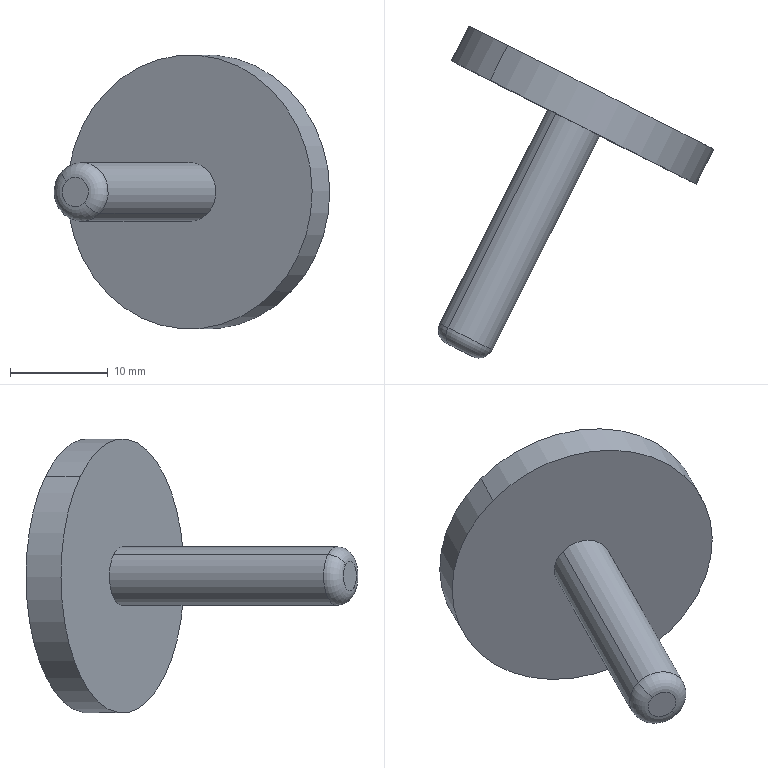Component | SolidWorks | Part15-1 | 2 solids | 10 faces | box 28.16 x 33.93 x 28 mm | volume 3190 mm3 | cylinder 4 | plane 4 | torus 2 | commonest cylinder face diameters 6 x2 28 x2
STEP:
#1=COLOUR_RGB('',0.7922,0.8196,0.9333);
#2=FILL_AREA_STYLE_COLOUR('',#1);
#3=FILL_AREA_STYLE('',(#2));
#4=SURFACE_STYLE_FILL_AREA(#3);
#5=SURFACE_SIDE_STYLE('',(#4));
#6=SURFACE_STYLE_USAGE(.BOTH.,#5);
#7=PRESENTATION_STYLE_ASSIGNMENT((#6));
#8=CARTESIAN_POINT('',(1.257,1.983,-0.3626));
#9=VERTEX_POINT('',#8);
#10=CARTESIAN_POINT('',(0.5828,2.322,0.4413));
#11=VERTEX_POINT('',#10);
#12=CARTESIAN_POINT('',(0.9197,2.152,0.03937));
#13=DIRECTION('',(0.4496,0.8932,-0.));
#14=DIRECTION('',(0.6112,-0.3076,-0.7292));
#15=AXIS2_PLACEMENT_3D('',#12,#13,#14);
#16=CIRCLE('',#15,0.5512);
#17=EDGE_CURVE('',#9,#11,#16,.T.);
#18=ORIENTED_EDGE('',*,*,#17,.F.);
#19=CARTESIAN_POINT('',(1.186,1.842,-0.3626));
#20=VERTEX_POINT('',#19);
#21=CARTESIAN_POINT('',(1.257,1.983,-0.3626));
#22=DIRECTION('',(-0.4496,-0.8932,0.));
#23=VECTOR('',#22,39.37);
#24=LINE('',#21,#23);
#25=EDGE_CURVE('',#9,#20,#24,.T.);
#26=ORIENTED_EDGE('',*,*,#25,.T.);
#27=CARTESIAN_POINT('',(0.512,2.181,0.4413));
#28=VERTEX_POINT('',#27);
#29=CARTESIAN_POINT('',(0.8489,2.012,0.03937));
#30=DIRECTION('',(0.4496,0.8932,-0.));
#31=DIRECTION('',(0.6112,-0.3076,-0.7292));
#32=AXIS2_PLACEMENT_3D('',#29,#30,#31);
#33=CIRCLE('',#32,0.5512);
#34=EDGE_CURVE('',#20,#28,#33,.T.);
#35=ORIENTED_EDGE('',*,*,#34,.T.);
#36=CARTESIAN_POINT('',(0.5828,2.322,0.4413));
#37=DIRECTION('',(-0.4496,-0.8932,0.));
#38=VECTOR('',#37,39.37);
#39=LINE('',#36,#38);
#40=EDGE_CURVE('',#11,#28,#39,.T.);
#41=ORIENTED_EDGE('',*,*,#40,.F.);
#42=EDGE_LOOP('',(#18,#26,#35,#41));
#43=FACE_OUTER_BOUND('',#42,.T.);
#44=CARTESIAN_POINT('',(0.9197,2.152,0.03937));
#45=DIRECTION('',(-0.4496,-0.8932,0.));
#46=DIRECTION('',(-0.6112,0.3076,0.7292));
#47=AXIS2_PLACEMENT_3D('',#44,#45,#46);
#48=CYLINDRICAL_SURFACE('',#47,0.5512);
#49=ADVANCED_FACE('',(#43),#48,.T.);
#50=CARTESIAN_POINT('',(0.8489,2.012,0.03937));
#51=DIRECTION('',(0.4496,0.8932,-0.));
#52=DIRECTION('',(0.6112,-0.3076,-0.7292));
#53=AXIS2_PLACEMENT_3D('',#50,#51,#52);
#54=CIRCLE('',#53,0.5512);
#55=EDGE_CURVE('',#28,#20,#54,.T.);
#56=ORIENTED_EDGE('',*,*,#55,.F.);
#57=ORIENTED_EDGE('',*,*,#34,.F.);
#58=EDGE_LOOP('',(#56,#57));
#59=FACE_OUTER_BOUND('',#58,.T.);
#60=CARTESIAN_POINT('',(0.8489,2.012,0.03937));
#61=DIRECTION('',(0.4496,0.8932,-0.));
#62=DIRECTION('',(0.6514,-0.3278,0.6843));
#63=AXIS2_PLACEMENT_3D('',#60,#61,#62);
#64=PLANE('',#63);
#65=ADVANCED_FACE('',(#59),#64,.F.);
#66=CARTESIAN_POINT('',(0.9197,2.152,0.03937));
#67=DIRECTION('',(0.4496,0.8932,-0.));
#68=DIRECTION('',(0.6112,-0.3076,-0.7292));
#69=AXIS2_PLACEMENT_3D('',#66,#67,#68);
#70=CIRCLE('',#69,0.5512);
#71=EDGE_CURVE('',#11,#9,#70,.T.);
#72=ORIENTED_EDGE('',*,*,#71,.T.);
#73=ORIENTED_EDGE('',*,*,#17,.T.);
#74=EDGE_LOOP('',(#72,#73));
#75=FACE_OUTER_BOUND('',#74,.T.);
#76=CARTESIAN_POINT('',(0.9197,2.152,0.03937));
#77=DIRECTION('',(0.4496,0.8932,-0.));
#78=DIRECTION('',(0.6514,-0.3278,0.6843));
#79=AXIS2_PLACEMENT_3D('',#76,#77,#78);
#80=PLANE('',#79);
#81=ADVANCED_FACE('',(#75),#80,.T.);
#82=ORIENTED_EDGE('',*,*,#25,.F.);
#83=ORIENTED_EDGE('',*,*,#71,.F.);
#84=ORIENTED_EDGE('',*,*,#40,.T.);
#85=ORIENTED_EDGE('',*,*,#55,.T.);
#86=EDGE_LOOP('',(#82,#83,#84,#85));
#87=FACE_OUTER_BOUND('',#86,.T.);
#88=CARTESIAN_POINT('',(0.9197,2.152,0.03937));
#89=DIRECTION('',(-0.4496,-0.8932,0.));
#90=DIRECTION('',(-0.6112,0.3076,0.7292));
#91=AXIS2_PLACEMENT_3D('',#88,#89,#90);
#92=CYLINDRICAL_SURFACE('',#91,0.5512);
#93=ADVANCED_FACE('',(#87),#92,.T.);
#94=CLOSED_SHELL('',(#49,#65,#81,#93));
#95=MANIFOLD_SOLID_BREP('',#94);
#96=STYLED_ITEM('',(#7),#95);
#97=PRESENTATION_LAYER_ASSIGNMENT('','',(#96));
#98=COLOUR_RGB('',0.7922,0.8196,0.9333);
#99=FILL_AREA_STYLE_COLOUR('',#98);
#100=FILL_AREA_STYLE('',(#99));
#101=SURFACE_STYLE_FILL_AREA(#100);
#102=SURFACE_SIDE_STYLE('',(#101));
#103=SURFACE_STYLE_USAGE(.BOTH.,#102);
#104=PRESENTATION_STYLE_ASSIGNMENT((#103));
#105=CARTESIAN_POINT('',(0.4874,1.114,-0.04676));
#106=VERTEX_POINT('',#105);
#107=CARTESIAN_POINT('',(0.343,1.186,0.1255));
#108=VERTEX_POINT('',#107);
#109=CARTESIAN_POINT('',(0.4152,1.15,0.03937));
#110=DIRECTION('',(0.4496,0.8932,-0.));
#111=DIRECTION('',(-0.6112,0.3076,0.7292));
#112=AXIS2_PLACEMENT_3D('',#109,#110,#111);
#113=CIRCLE('',#112,0.1181);
#114=EDGE_CURVE('',#106,#108,#113,.T.);
#115=ORIENTED_EDGE('',*,*,#114,.T.);
#116=CARTESIAN_POINT('',(0.7767,2.048,0.1255));
#117=VERTEX_POINT('',#116);
#118=CARTESIAN_POINT('',(0.3165,1.134,0.1255));
#119=DIRECTION('',(0.4496,0.8932,-0.));
#120=VECTOR('',#119,39.37);
#121=LINE('',#118,#120);
#122=EDGE_CURVE('',#108,#117,#121,.T.);
#123=ORIENTED_EDGE('',*,*,#122,.T.);
#124=CARTESIAN_POINT('',(0.9211,1.975,-0.04676));
#125=VERTEX_POINT('',#124);
#126=CARTESIAN_POINT('',(0.8489,2.012,0.03937));
#127=DIRECTION('',(-0.4496,-0.8932,0.));
#128=DIRECTION('',(-0.6112,0.3076,0.7292));
#129=AXIS2_PLACEMENT_3D('',#126,#127,#128);
#130=CIRCLE('',#129,0.1181);
#131=EDGE_CURVE('',#117,#125,#130,.T.);
#132=ORIENTED_EDGE('',*,*,#131,.T.);
#133=CARTESIAN_POINT('',(0.4609,1.061,-0.04676));
#134=DIRECTION('',(0.4496,0.8932,-0.));
#135=VECTOR('',#134,39.37);
#136=LINE('',#133,#135);
#137=EDGE_CURVE('',#106,#125,#136,.T.);
#138=ORIENTED_EDGE('',*,*,#137,.F.);
#139=EDGE_LOOP('',(#115,#123,#132,#138));
#140=FACE_OUTER_BOUND('',#139,.T.);
#141=CARTESIAN_POINT('',(0.3887,1.097,0.03937));
#142=DIRECTION('',(0.4496,0.8932,-0.));
#143=DIRECTION('',(0.6112,-0.3076,-0.7292));
#144=AXIS2_PLACEMENT_3D('',#141,#142,#143);
#145=CYLINDRICAL_SURFACE('',#144,0.1181);
#146=ADVANCED_FACE('',(#140),#145,.T.);
#147=ORIENTED_EDGE('',*,*,#114,.F.);
#148=CARTESIAN_POINT('',(0.4248,1.079,-0.003695));
#149=VERTEX_POINT('',#148);
#150=CARTESIAN_POINT('',(0.4513,1.132,-0.003695));
#151=DIRECTION('',(-0.6514,0.3278,-0.6843));
#152=DIRECTION('',(-0.7243,0.,0.6895));
#153=AXIS2_PLACEMENT_3D('',#150,#151,#152);
#154=CIRCLE('',#153,0.05906);
#155=EDGE_CURVE('',#106,#149,#154,.T.);
#156=ORIENTED_EDGE('',*,*,#155,.T.);
#157=CARTESIAN_POINT('',(0.3526,1.115,0.08243));
#158=VERTEX_POINT('',#157);
#159=CARTESIAN_POINT('',(0.3887,1.097,0.03937));
#160=DIRECTION('',(-0.4496,-0.8932,0.));
#161=DIRECTION('',(-0.6112,0.3076,0.7292));
#162=AXIS2_PLACEMENT_3D('',#159,#160,#161);
#163=CIRCLE('',#162,0.05906);
#164=EDGE_CURVE('',#158,#149,#163,.T.);
#165=ORIENTED_EDGE('',*,*,#164,.F.);
#166=CARTESIAN_POINT('',(0.3791,1.168,0.08243));
#167=DIRECTION('',(0.6514,-0.3278,0.6843));
#168=DIRECTION('',(0.7243,0.,-0.6895));
#169=AXIS2_PLACEMENT_3D('',#166,#167,#168);
#170=CIRCLE('',#169,0.05906);
#171=EDGE_CURVE('',#108,#158,#170,.T.);
#172=ORIENTED_EDGE('',*,*,#171,.F.);
#173=EDGE_LOOP('',(#147,#156,#165,#172));
#174=FACE_OUTER_BOUND('',#173,.T.);
#175=CARTESIAN_POINT('',(0.4152,1.15,0.03937));
#176=DIRECTION('',(-0.4496,-0.8932,0.));
#177=DIRECTION('',(-0.6112,0.3076,0.7292));
#178=AXIS2_PLACEMENT_3D('',#175,#176,#177);
#179=TOROIDAL_SURFACE('',#178,0.05906,0.05906);
#180=ADVANCED_FACE('',(#174),#179,.T.);
#181=ORIENTED_EDGE('',*,*,#155,.F.);
#182=CARTESIAN_POINT('',(0.4152,1.15,0.03937));
#183=DIRECTION('',(0.4496,0.8932,-0.));
#184=DIRECTION('',(-0.6112,0.3076,0.7292));
#185=AXIS2_PLACEMENT_3D('',#182,#183,#184);
#186=CIRCLE('',#185,0.1181);
#187=EDGE_CURVE('',#108,#106,#186,.T.);
#188=ORIENTED_EDGE('',*,*,#187,.F.);
#189=ORIENTED_EDGE('',*,*,#171,.T.);
#190=CARTESIAN_POINT('',(0.3887,1.097,0.03937));
#191=DIRECTION('',(-0.4496,-0.8932,0.));
#192=DIRECTION('',(-0.6112,0.3076,0.7292));
#193=AXIS2_PLACEMENT_3D('',#190,#191,#192);
#194=CIRCLE('',#193,0.05906);
#195=EDGE_CURVE('',#149,#158,#194,.T.);
#196=ORIENTED_EDGE('',*,*,#195,.F.);
#197=EDGE_LOOP('',(#181,#188,#189,#196));
#198=FACE_OUTER_BOUND('',#197,.T.);
#199=CARTESIAN_POINT('',(0.4152,1.15,0.03937));
#200=DIRECTION('',(-0.4496,-0.8932,0.));
#201=DIRECTION('',(-0.6112,0.3076,0.7292));
#202=AXIS2_PLACEMENT_3D('',#199,#200,#201);
#203=TOROIDAL_SURFACE('',#202,0.05906,0.05906);
#204=ADVANCED_FACE('',(#198),#203,.T.);
#205=CARTESIAN_POINT('',(0.8489,2.012,0.03937));
#206=DIRECTION('',(-0.4496,-0.8932,0.));
#207=DIRECTION('',(-0.6112,0.3076,0.7292));
#208=AXIS2_PLACEMENT_3D('',#205,#206,#207);
#209=CIRCLE('',#208,0.1181);
#210=EDGE_CURVE('',#125,#117,#209,.T.);
#211=ORIENTED_EDGE('',*,*,#210,.F.);
#212=ORIENTED_EDGE('',*,*,#131,.F.);
#213=EDGE_LOOP('',(#211,#212));
#214=FACE_OUTER_BOUND('',#213,.T.);
#215=CARTESIAN_POINT('',(0.8489,2.012,0.03937));
#216=DIRECTION('',(-0.4496,-0.8932,0.));
#217=DIRECTION('',(0.6112,-0.3076,-0.7292));
#218=AXIS2_PLACEMENT_3D('',#215,#216,#217);
#219=PLANE('',#218);
#220=ADVANCED_FACE('',(#214),#219,.F.);
#221=ORIENTED_EDGE('',*,*,#164,.T.);
#222=ORIENTED_EDGE('',*,*,#195,.T.);
#223=EDGE_LOOP('',(#221,#222));
#224=FACE_OUTER_BOUND('',#223,.T.);
#225=CARTESIAN_POINT('',(0.3887,1.097,0.03937));
#226=DIRECTION('',(-0.4496,-0.8932,0.));
#227=DIRECTION('',(0.6112,-0.3076,-0.7292));
#228=AXIS2_PLACEMENT_3D('',#225,#226,#227);
#229=PLANE('',#228);
#230=ADVANCED_FACE('',(#224),#229,.T.);
#231=ORIENTED_EDGE('',*,*,#122,.F.);
#232=ORIENTED_EDGE('',*,*,#187,.T.);
#233=ORIENTED_EDGE('',*,*,#137,.T.);
#234=ORIENTED_EDGE('',*,*,#210,.T.);
#235=EDGE_LOOP('',(#231,#232,#233,#234));
#236=FACE_OUTER_BOUND('',#235,.T.);
#237=CARTESIAN_POINT('',(0.3887,1.097,0.03937));
#238=DIRECTION('',(0.4496,0.8932,-0.));
#239=DIRECTION('',(0.6112,-0.3076,-0.7292));
#240=AXIS2_PLACEMENT_3D('',#237,#238,#239);
#241=CYLINDRICAL_SURFACE('',#240,0.1181);
#242=ADVANCED_FACE('',(#236),#241,.T.);
#243=CLOSED_SHELL('',(#146,#180,#204,#220,#230,#242));
#244=MANIFOLD_SOLID_BREP('',#243);
#245=STYLED_ITEM('',(#104),#244);
#246=(LENGTH_UNIT()NAMED_UNIT(*)SI_UNIT($,.METRE.));
#247=LENGTH_MEASURE_WITH_UNIT(LENGTH_MEASURE(0.0254),#246);
#248=DIMENSIONAL_EXPONENTS(1.,0.,0.,0.,0.,0.,0.);
#249=(CONVERSION_BASED_UNIT('',#247)LENGTH_UNIT()NAMED_UNIT(#248));
#250=UNCERTAINTY_MEASURE_WITH_UNIT(LENGTH_MEASURE(0.00001),#249,'','');
#251=(NAMED_UNIT(*)PLANE_ANGLE_UNIT()SI_UNIT($,.RADIAN.));
#252=(NAMED_UNIT(*)SI_UNIT($,.STERADIAN.)SOLID_ANGLE_UNIT());
#253=(GEOMETRIC_REPRESENTATION_CONTEXT(3)GLOBAL_UNCERTAINTY_ASSIGNED_CONTEXT((#250))GLOBAL_UNIT_ASSIGNED_CONTEXT((#249,#251,#252))REPRESENTATION_CONTEXT('',''));
#254=MECHANICAL_DESIGN_GEOMETRIC_PRESENTATION_REPRESENTATION('',(#245),#253);
#255=(LENGTH_UNIT()NAMED_UNIT(*)SI_UNIT($,.METRE.));
#256=LENGTH_MEASURE_WITH_UNIT(LENGTH_MEASURE(0.0254),#255);
#257=DIMENSIONAL_EXPONENTS(1.,0.,0.,0.,0.,0.,0.);
#258=(CONVERSION_BASED_UNIT('',#256)LENGTH_UNIT()NAMED_UNIT(#257));
#259=UNCERTAINTY_MEASURE_WITH_UNIT(LENGTH_MEASURE(0.00001),#258,'','');
#260=(NAMED_UNIT(*)PLANE_ANGLE_UNIT()SI_UNIT($,.RADIAN.));
#261=(NAMED_UNIT(*)SI_UNIT($,.STERADIAN.)SOLID_ANGLE_UNIT());
#262=(GEOMETRIC_REPRESENTATION_CONTEXT(3)GLOBAL_UNCERTAINTY_ASSIGNED_CONTEXT((#259))GLOBAL_UNIT_ASSIGNED_CONTEXT((#258,#260,#261))REPRESENTATION_CONTEXT('',''));
#263=MECHANICAL_DESIGN_GEOMETRIC_PRESENTATION_REPRESENTATION('',(#96),#262);
#264=CARTESIAN_POINT('',(0.,0.,0.));
#265=DIRECTION('',(0.,0.,1.));
#266=DIRECTION('',(1.,0.,0.));
#267=AXIS2_PLACEMENT_3D('',#264,#265,#266);
#268=(LENGTH_UNIT()NAMED_UNIT(*)SI_UNIT($,.METRE.));
#269=LENGTH_MEASURE_WITH_UNIT(LENGTH_MEASURE(0.0254),#268);
#270=DIMENSIONAL_EXPONENTS(1.,0.,0.,0.,0.,0.,0.);
#271=(CONVERSION_BASED_UNIT('',#269)LENGTH_UNIT()NAMED_UNIT(#270));
#272=UNCERTAINTY_MEASURE_WITH_UNIT(LENGTH_MEASURE(0.00001),#271,'','');
#273=(NAMED_UNIT(*)PLANE_ANGLE_UNIT()SI_UNIT($,.RADIAN.));
#274=(NAMED_UNIT(*)SI_UNIT($,.STERADIAN.)SOLID_ANGLE_UNIT());
#275=(GEOMETRIC_REPRESENTATION_CONTEXT(3)GLOBAL_UNCERTAINTY_ASSIGNED_CONTEXT((#272))GLOBAL_UNIT_ASSIGNED_CONTEXT((#271,#273,#274))REPRESENTATION_CONTEXT('',''));
#276=ADVANCED_BREP_SHAPE_REPRESENTATION('',(#244,#95,#267),#275);
#277=PRESENTATION_LAYER_ASSIGNMENT('','',(#245));